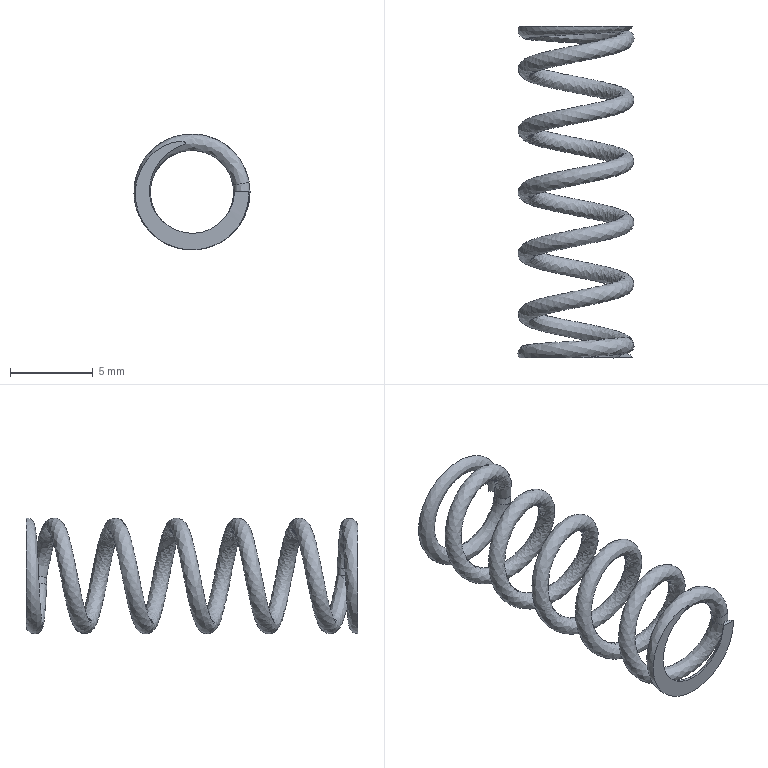Component | NX | SPRING | 1 solid | 9 faces | volume 99 mm3 | spline 5 | plane 4